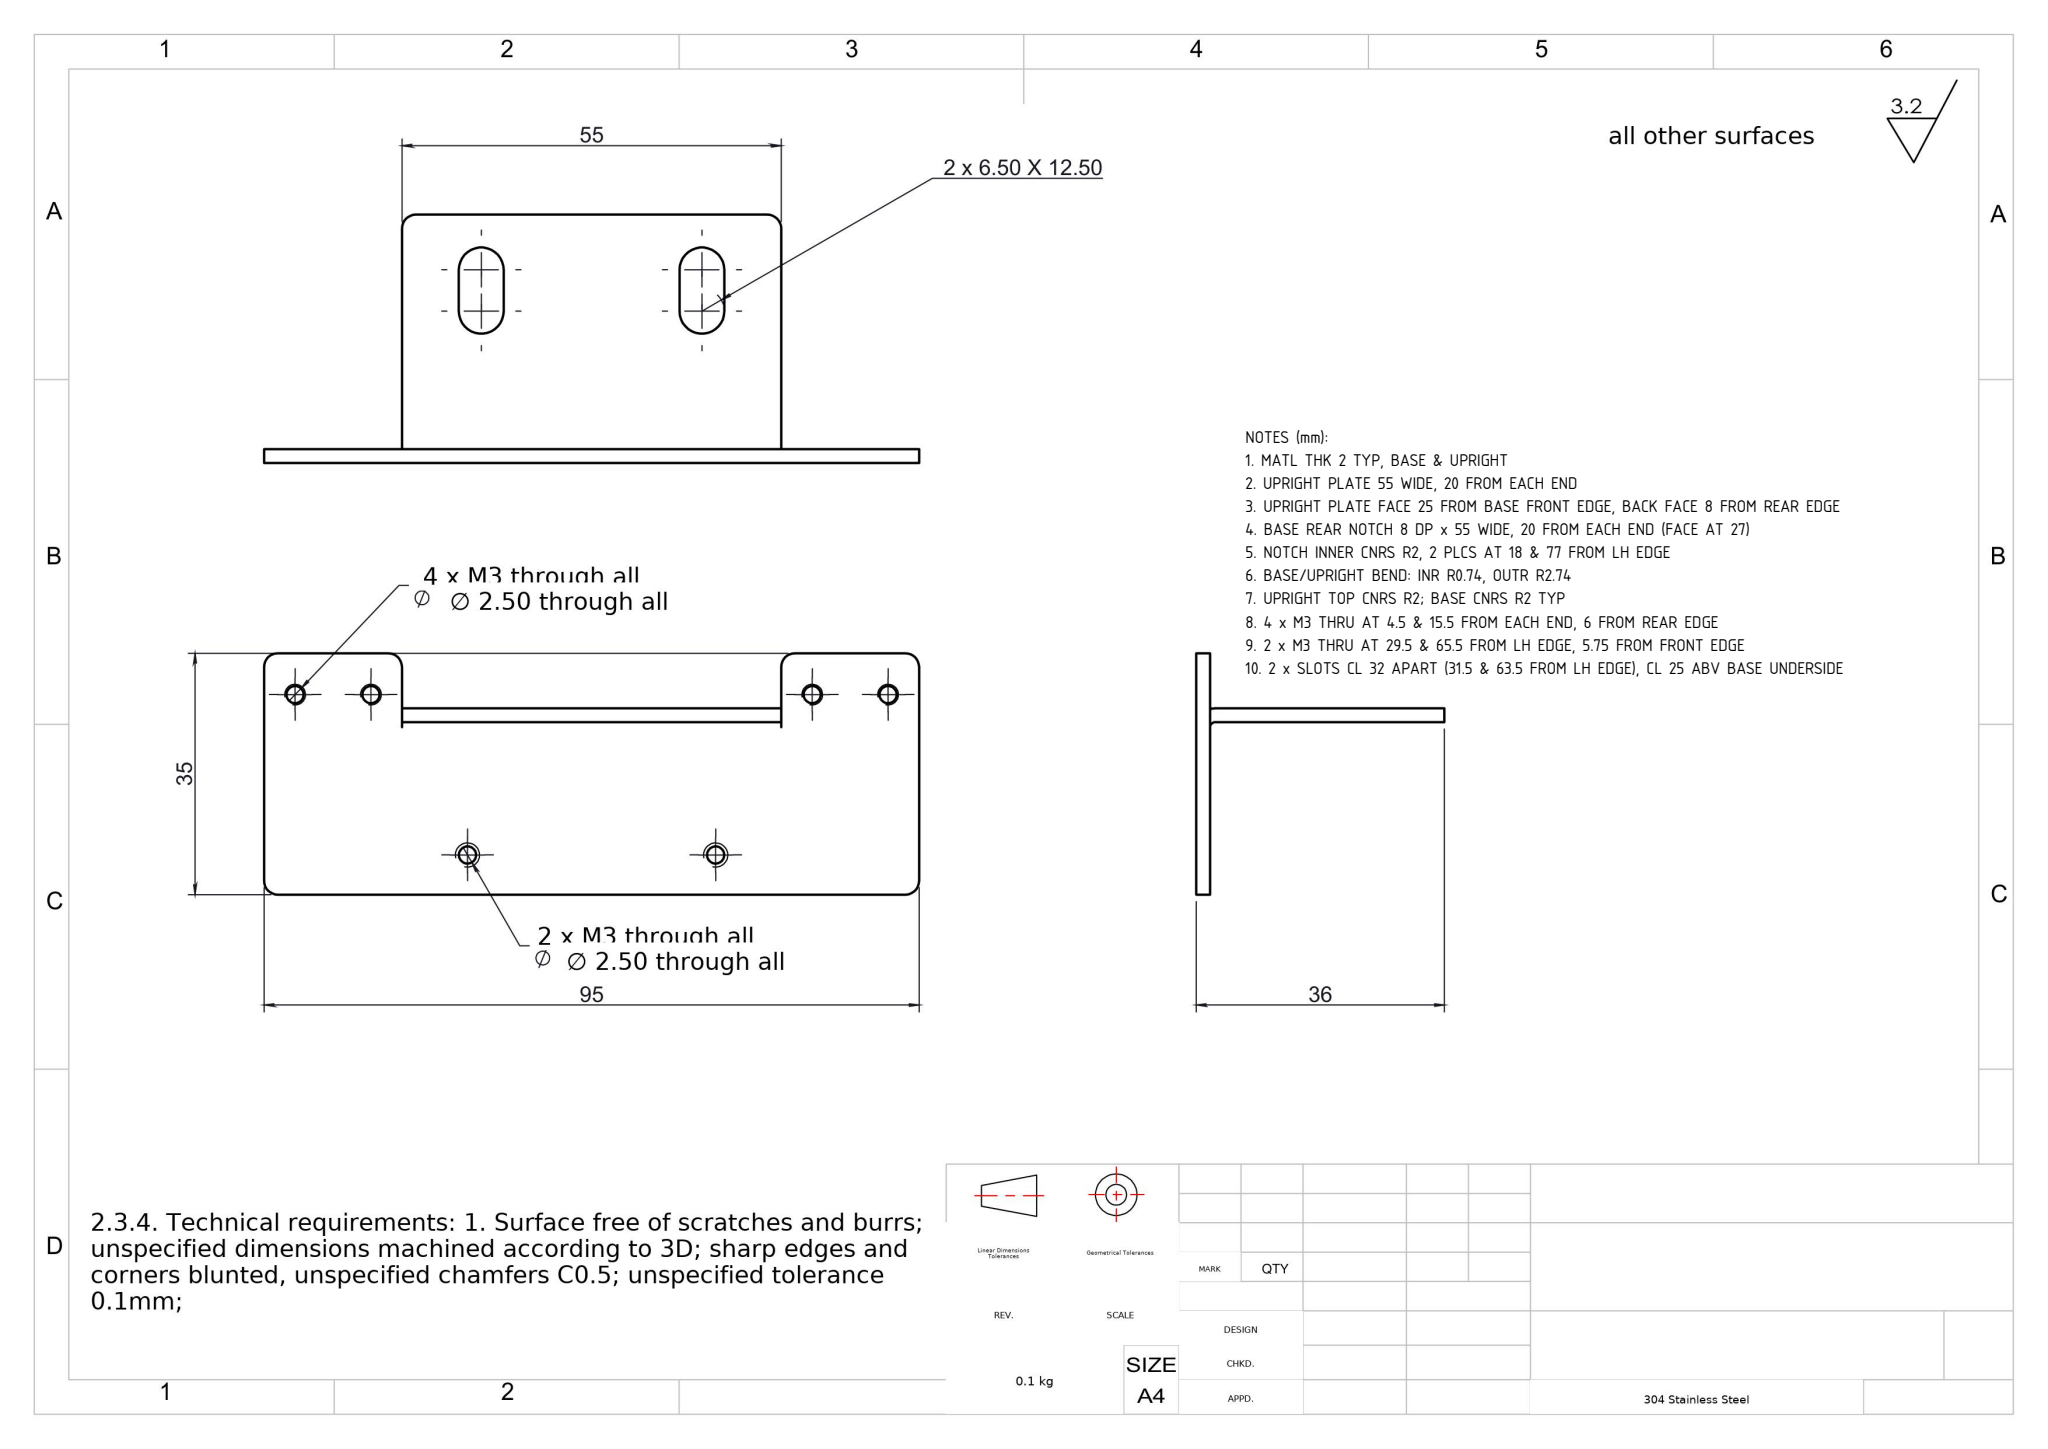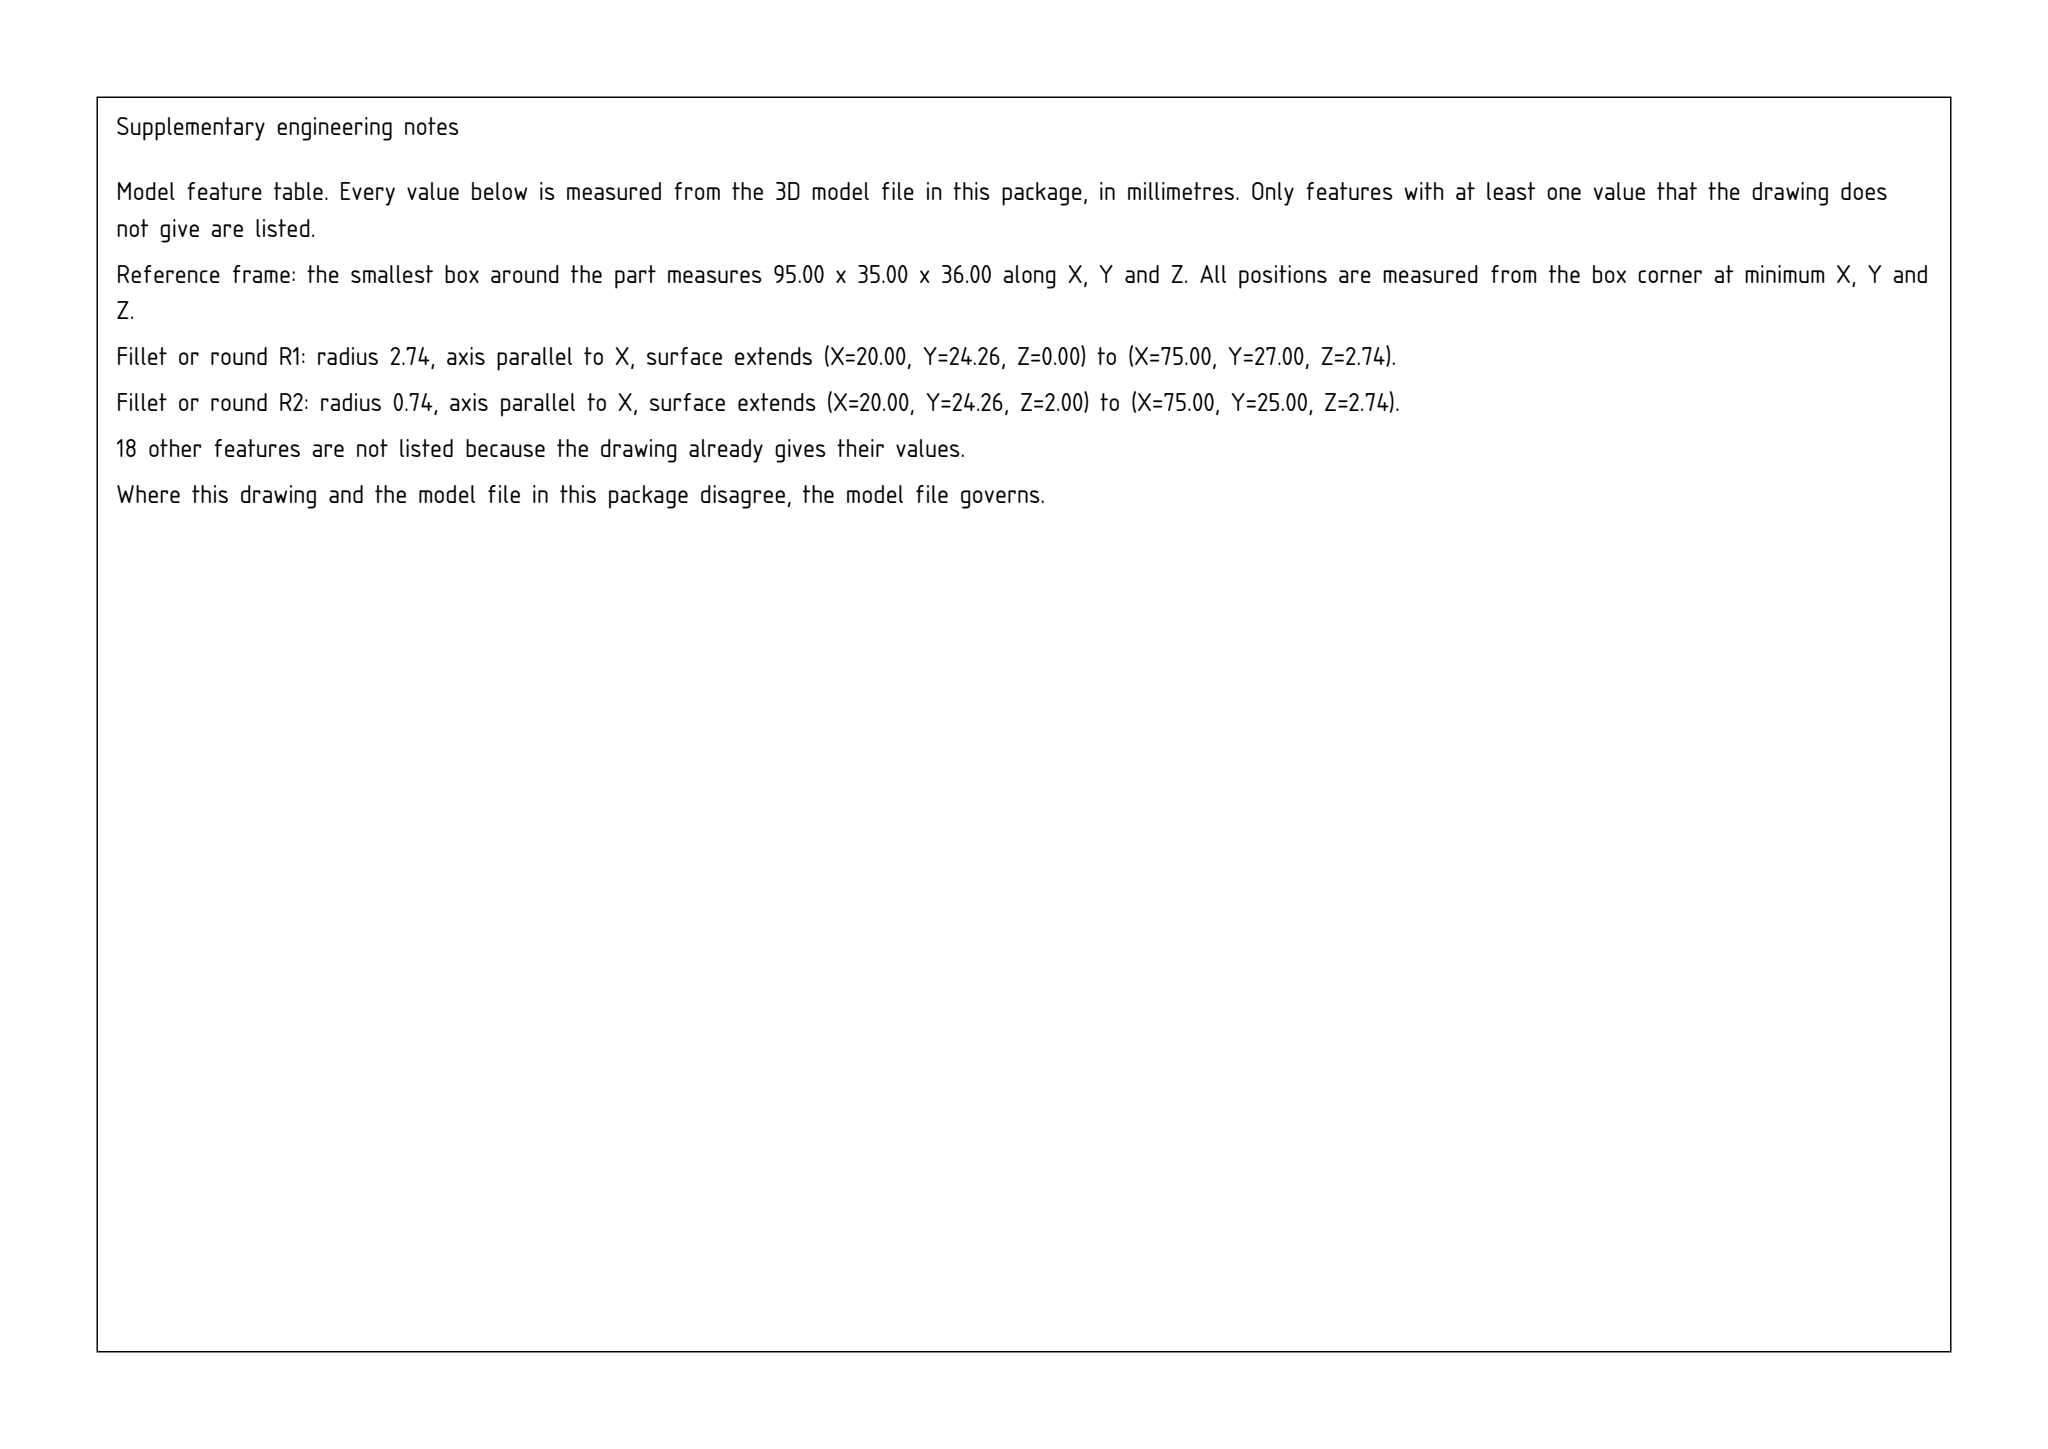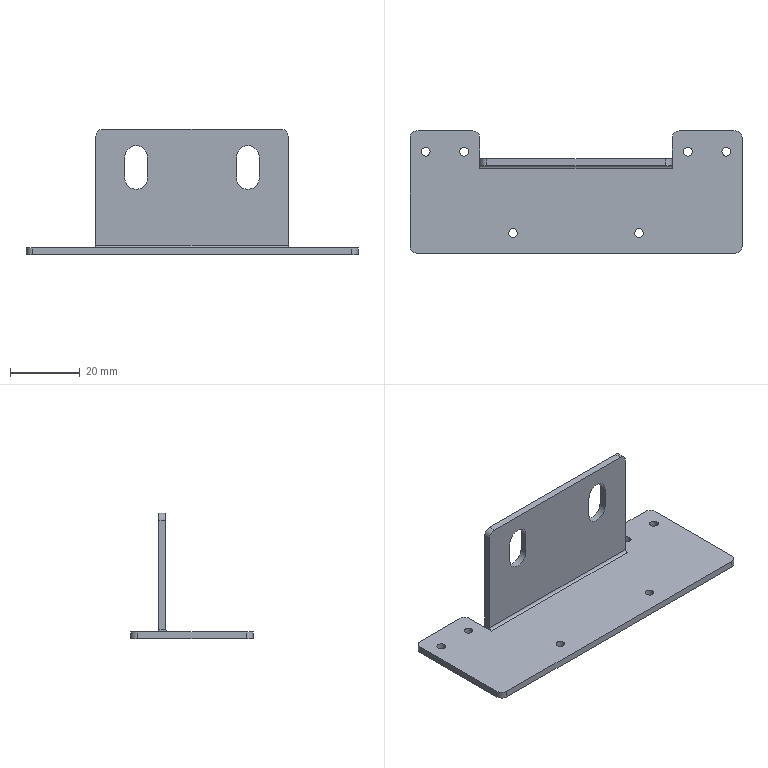Part | SolidWorks | mm | 1 solid | 48 faces | box 95 x 35 x 36 mm | volume 9067 mm3 | cylinder 28 | plane 20 | commonest cylinder face diameters 2.5 x12 4 x8 6.5 x6 5.473 x1 1.473 x1
Drawing notes:
MATL THK 2 TYP, BASE & UPRIGHT | from the solid: z planes 0/2 (base); y planes 25/27 (upright)
UPRIGHT PLATE 55 WIDE, 20 FROM EACH END | from the solid: x planes 20 & 75 = 55 wide; 95-75=20
UPRIGHT PLATE FACE 25 FROM BASE FRONT EDGE, BACK FACE 8 FROM REAR EDGE | from the solid: y planes 25 & 27; base y 0-35
BASE REAR NOTCH 8 DP x 55 WIDE, 20 FROM EACH END (FACE AT 27) | from the solid: y plane 27 between x planes 20 & 75; base y 0-35
NOTCH INNER CNRS R2, 2 PLCS AT 18 & 77 FROM LH EDGE | from the solid: Ø4.0 z-axis cyls at (18,33) & (77,33), len 2
BASE/UPRIGHT BEND: INR R0.74, OUTR R2.74 | from the solid: x-axis cyls Ø1.473 & Ø5.473 at (y24.26,z2.74), L=55
UPRIGHT TOP CNRS R2; BASE CNRS R2 TYP | from the solid: Ø4 y-cyls at (22,34),(73,34); Ø4 z-cyls at base cnrs
4 x M3 THRU AT 4.5 & 15.5 FROM EACH END, 6 FROM REAR EDGE | from the solid: Ø2.5 z-holes x=4.5,15.5,79.5,90.5; y=29 of 35
2 x M3 THRU AT 29.5 & 65.5 FROM LH EDGE, 5.75 FROM FRONT EDGE | from the solid: Ø2.5 z-holes at (29.5,5.75) & (65.5,5.75)
2 x SLOTS CL 32 APART (31.5 & 63.5 FROM LH EDGE), CL 25 ABV BASE UNDERSIDE | from the solid: Ø6.5 y-holes x=31.5 & 63.5, z=22 & 28 (CL z=25)